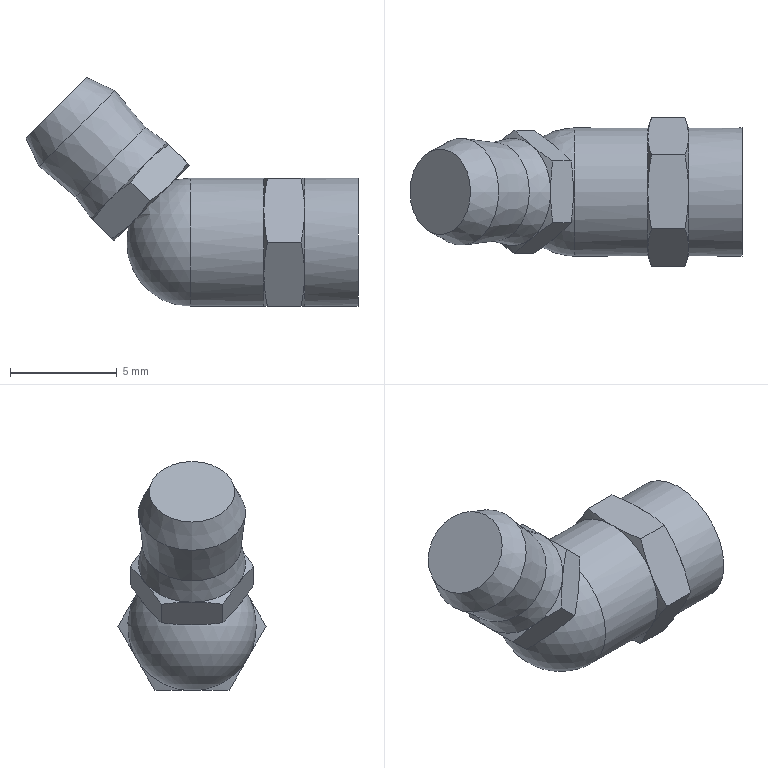Component | NX | SLIDER_3 | 1 solid | 45 faces | volume 398 mm3 | cone 27 | plane 15 | cylinder 2 | sphere 1 | commonest cylinder face diameters 6 x2